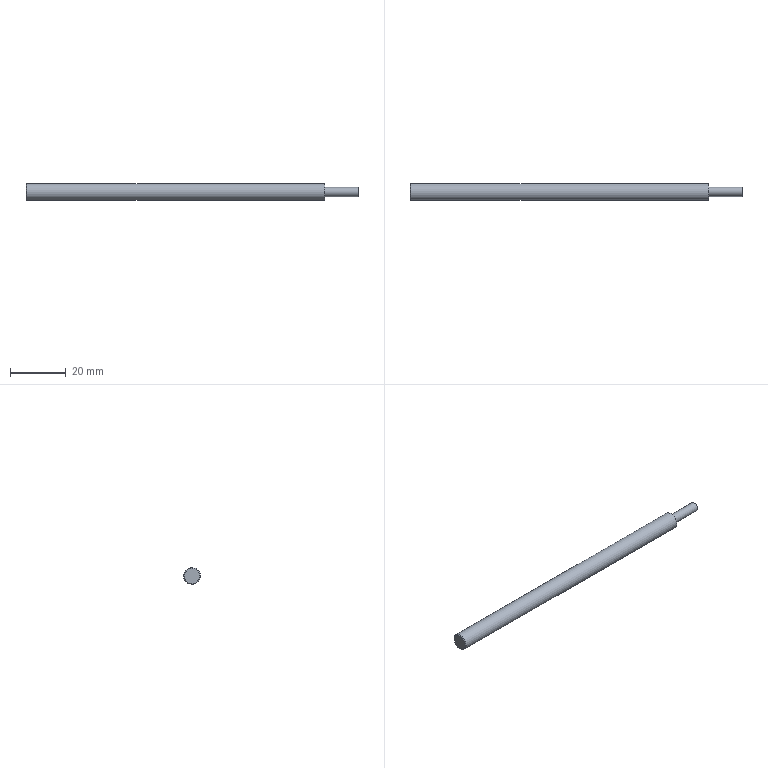Component | NX | PISTON_ROD | 1 solid | 6 faces | box 119 x 6 x 6 mm | volume 3127 mm3 | plane 3 | cylinder 2 | cone 1 | commonest cylinder face diameters 6 x1 3.3 x1
STEP:
#1=CARTESIAN_POINT('',(0.,0.,0.));
#2=DIRECTION('',(0.,0.,1.));
#3=DIRECTION('',(1.,0.,0.));
#4=AXIS2_PLACEMENT_3D('',#1,#2,#3);
#5=CARTESIAN_POINT('',(301.474,86.751,111.081));
#6=VERTEX_POINT('',#5);
#7=CARTESIAN_POINT('',(301.474,89.5,111.));
#8=DIRECTION('',(-1.,0.,0.));
#9=DIRECTION('',(0.,-0.9996,0.02941));
#10=AXIS2_PLACEMENT_3D('',#7,#8,#9);
#11=CIRCLE('',#10,2.75);
#12=CARTESIAN_POINT('',(301.474,89.5,111.));
#13=DIRECTION('',(-1.,0.,0.));
#14=DIRECTION('',(0.,-0.9996,0.02941));
#15=AXIS2_PLACEMENT_3D('',#12,#13,#14);
#16=PLANE('',#15);
#17=CARTESIAN_POINT('',(0.,0.));
#18=DIRECTION('',(1.,0.));
#19=AXIS2_PLACEMENT_2D('',#17,#18);
#20=CIRCLE('',#19,2.75);
#21=(GEOMETRIC_REPRESENTATION_CONTEXT(2)PARAMETRIC_REPRESENTATION_CONTEXT()REPRESENTATION_CONTEXT('',''));
#22=DEFINITIONAL_REPRESENTATION('',(#20),#21);
#23=PCURVE('',#16,#22);
#24=CARTESIAN_POINT('',(301.724,89.5,111.));
#25=DIRECTION('',(1.,0.,0.));
#26=DIRECTION('',(0.,0.9996,-0.02941));
#27=AXIS2_PLACEMENT_3D('',#24,#25,#26);
#28=CONICAL_SURFACE('',#27,3.,0.7854);
#29=CARTESIAN_POINT('',(9.425,-0.25));
#30=DIRECTION('',(-1.,0.));
#31=VECTOR('',#30,1.);
#32=LINE('',#29,#31);
#33=(GEOMETRIC_REPRESENTATION_CONTEXT(2)PARAMETRIC_REPRESENTATION_CONTEXT()REPRESENTATION_CONTEXT('',''));
#34=DEFINITIONAL_REPRESENTATION('',(#32),#33);
#35=PCURVE('',#28,#34);
#36=SURFACE_CURVE('',#11,(#23,#35),.PCURVE_S1.);
#37=EDGE_CURVE('',#6,#6,#36,.T.);
#38=ORIENTED_EDGE('',*,*,#37,.T.);
#39=EDGE_LOOP('',(#38));
#40=FACE_BOUND('',#39,.T.);
#41=ADVANCED_FACE('',(#40),#16,.T.);
#42=CARTESIAN_POINT('',(408.474,91.149,110.951));
#43=VERTEX_POINT('',#42);
#44=CARTESIAN_POINT('',(408.474,89.5,111.));
#45=DIRECTION('',(1.,0.,0.));
#46=DIRECTION('',(0.,0.9996,-0.02941));
#47=AXIS2_PLACEMENT_3D('',#44,#45,#46);
#48=CIRCLE('',#47,1.65);
#49=CARTESIAN_POINT('',(408.474,89.5,111.));
#50=DIRECTION('',(1.,0.,0.));
#51=DIRECTION('',(0.,0.9996,-0.02941));
#52=AXIS2_PLACEMENT_3D('',#49,#50,#51);
#53=PLANE('',#52);
#54=CARTESIAN_POINT('',(0.,0.));
#55=DIRECTION('',(1.,0.));
#56=AXIS2_PLACEMENT_2D('',#54,#55);
#57=CIRCLE('',#56,1.65);
#58=(GEOMETRIC_REPRESENTATION_CONTEXT(2)PARAMETRIC_REPRESENTATION_CONTEXT()REPRESENTATION_CONTEXT('',''));
#59=DEFINITIONAL_REPRESENTATION('',(#57),#58);
#60=PCURVE('',#53,#59);
#61=CARTESIAN_POINT('',(408.474,89.5,111.));
#62=DIRECTION('',(1.,0.,0.));
#63=DIRECTION('',(0.,0.9996,-0.02941));
#64=AXIS2_PLACEMENT_3D('',#61,#62,#63);
#65=CYLINDRICAL_SURFACE('',#64,1.65);
#66=CARTESIAN_POINT('',(0.,0.));
#67=DIRECTION('',(1.,0.));
#68=VECTOR('',#67,1.);
#69=LINE('',#66,#68);
#70=(GEOMETRIC_REPRESENTATION_CONTEXT(2)PARAMETRIC_REPRESENTATION_CONTEXT()REPRESENTATION_CONTEXT('',''));
#71=DEFINITIONAL_REPRESENTATION('',(#69),#70);
#72=PCURVE('',#65,#71);
#73=SURFACE_CURVE('',#48,(#60,#72),.PCURVE_S1.);
#74=EDGE_CURVE('',#43,#43,#73,.T.);
#75=ORIENTED_EDGE('',*,*,#74,.F.);
#76=EDGE_LOOP('',(#75));
#77=FACE_BOUND('',#76,.T.);
#78=CARTESIAN_POINT('',(408.474,86.501,111.088));
#79=VERTEX_POINT('',#78);
#80=CARTESIAN_POINT('',(408.474,89.5,111.));
#81=DIRECTION('',(-1.,0.,0.));
#82=DIRECTION('',(0.,-0.9996,0.02941));
#83=AXIS2_PLACEMENT_3D('',#80,#81,#82);
#84=CIRCLE('',#83,3.);
#85=CARTESIAN_POINT('',(-3.,-0.));
#86=CARTESIAN_POINT('',(-3.,5.196));
#87=CARTESIAN_POINT('',(1.5,2.598));
#88=CARTESIAN_POINT('',(6.,0.));
#89=CARTESIAN_POINT('',(1.5,-2.598));
#90=CARTESIAN_POINT('',(-3.,-5.196));
#91=CARTESIAN_POINT('',(-3.,-0.));
#92=(BOUNDED_CURVE()B_SPLINE_CURVE(2,(#85,#86,#87,#88,#89,#90,#91),.UNSPECIFIED.,.T.,.F.)B_SPLINE_CURVE_WITH_KNOTS((1,2,2,2,2,1),(-2.094,0.,2.094,4.189,6.283,8.378),.UNSPECIFIED.)CURVE()GEOMETRIC_REPRESENTATION_ITEM()RATIONAL_B_SPLINE_CURVE((1.,0.5,1.,0.5,1.,0.5,1.))REPRESENTATION_ITEM(''));
#93=(GEOMETRIC_REPRESENTATION_CONTEXT(2)PARAMETRIC_REPRESENTATION_CONTEXT()REPRESENTATION_CONTEXT('',''));
#94=DEFINITIONAL_REPRESENTATION('',(#92),#93);
#95=PCURVE('',#53,#94);
#96=CARTESIAN_POINT('',(408.474,89.5,111.));
#97=DIRECTION('',(-1.,0.,0.));
#98=DIRECTION('',(0.,-0.9996,0.02941));
#99=AXIS2_PLACEMENT_3D('',#96,#97,#98);
#100=CYLINDRICAL_SURFACE('',#99,3.);
#101=CARTESIAN_POINT('',(0.,0.));
#102=DIRECTION('',(1.,0.));
#103=VECTOR('',#102,1.);
#104=LINE('',#101,#103);
#105=(GEOMETRIC_REPRESENTATION_CONTEXT(2)PARAMETRIC_REPRESENTATION_CONTEXT()REPRESENTATION_CONTEXT('',''));
#106=DEFINITIONAL_REPRESENTATION('',(#104),#105);
#107=PCURVE('',#100,#106);
#108=SURFACE_CURVE('',#84,(#95,#107),.PCURVE_S1.);
#109=EDGE_CURVE('',#79,#79,#108,.T.);
#110=ORIENTED_EDGE('',*,*,#109,.F.);
#111=EDGE_LOOP('',(#110));
#112=FACE_BOUND('',#111,.T.);
#113=ADVANCED_FACE('',(#77,#112),#53,.T.);
#114=CARTESIAN_POINT('',(301.724,86.501,111.088));
#115=VERTEX_POINT('',#114);
#116=CARTESIAN_POINT('',(301.724,89.5,111.));
#117=DIRECTION('',(1.,0.,0.));
#118=DIRECTION('',(0.,-0.9996,0.02941));
#119=AXIS2_PLACEMENT_3D('',#116,#117,#118);
#120=CIRCLE('',#119,3.);
#121=CARTESIAN_POINT('',(6.283,106.75));
#122=DIRECTION('',(-1.,0.));
#123=VECTOR('',#122,1.);
#124=LINE('',#121,#123);
#125=(GEOMETRIC_REPRESENTATION_CONTEXT(2)PARAMETRIC_REPRESENTATION_CONTEXT()REPRESENTATION_CONTEXT('',''));
#126=DEFINITIONAL_REPRESENTATION('',(#124),#125);
#127=PCURVE('',#100,#126);
#128=CARTESIAN_POINT('',(3.142,0.));
#129=DIRECTION('',(1.,0.));
#130=VECTOR('',#129,1.);
#131=LINE('',#128,#130);
#132=(GEOMETRIC_REPRESENTATION_CONTEXT(2)PARAMETRIC_REPRESENTATION_CONTEXT()REPRESENTATION_CONTEXT('',''));
#133=DEFINITIONAL_REPRESENTATION('',(#131),#132);
#134=PCURVE('',#28,#133);
#135=SURFACE_CURVE('',#120,(#127,#134),.PCURVE_S1.);
#136=EDGE_CURVE('',#115,#115,#135,.T.);
#137=ORIENTED_EDGE('',*,*,#136,.T.);
#138=CARTESIAN_POINT('',(408.474,86.501,111.088));
#139=CARTESIAN_POINT('',(301.724,86.501,111.088));
#140=B_SPLINE_CURVE_WITH_KNOTS('',1,(#138,#139),.UNSPECIFIED.,.F.,.F.,(2,2),(0.,106.75),.PIECEWISE_BEZIER_KNOTS.);
#141=CARTESIAN_POINT('',(0.,0.));
#142=DIRECTION('',(0.,1.));
#143=VECTOR('',#142,1.);
#144=LINE('',#141,#143);
#145=(GEOMETRIC_REPRESENTATION_CONTEXT(2)PARAMETRIC_REPRESENTATION_CONTEXT()REPRESENTATION_CONTEXT('',''));
#146=DEFINITIONAL_REPRESENTATION('',(#144),#145);
#147=PCURVE('',#100,#146);
#148=CARTESIAN_POINT('',(6.283,0.));
#149=DIRECTION('',(0.,1.));
#150=VECTOR('',#149,1.);
#151=LINE('',#148,#150);
#152=(GEOMETRIC_REPRESENTATION_CONTEXT(2)PARAMETRIC_REPRESENTATION_CONTEXT()REPRESENTATION_CONTEXT('',''));
#153=DEFINITIONAL_REPRESENTATION('',(#151),#152);
#154=PCURVE('',#100,#153);
#155=SEAM_CURVE('',#140,(#147,#154),.PCURVE_S1.);
#156=EDGE_CURVE('',#79,#115,#155,.T.);
#157=ORIENTED_EDGE('',*,*,#156,.F.);
#158=ORIENTED_EDGE('',*,*,#109,.T.);
#159=ORIENTED_EDGE('',*,*,#156,.T.);
#160=EDGE_LOOP('',(#137,#157,#158,#159));
#161=FACE_BOUND('',#160,.T.);
#162=ADVANCED_FACE('',(#161),#100,.T.);
#163=CARTESIAN_POINT('',(420.474,91.149,110.951));
#164=VERTEX_POINT('',#163);
#165=CARTESIAN_POINT('',(420.474,89.5,111.));
#166=DIRECTION('',(1.,0.,0.));
#167=DIRECTION('',(0.,0.9996,-0.02941));
#168=AXIS2_PLACEMENT_3D('',#165,#166,#167);
#169=CIRCLE('',#168,1.65);
#170=CARTESIAN_POINT('',(420.474,89.5,111.));
#171=DIRECTION('',(1.,0.,0.));
#172=DIRECTION('',(0.,0.9996,-0.02941));
#173=AXIS2_PLACEMENT_3D('',#170,#171,#172);
#174=PLANE('',#173);
#175=CARTESIAN_POINT('',(0.,0.));
#176=DIRECTION('',(1.,0.));
#177=AXIS2_PLACEMENT_2D('',#175,#176);
#178=CIRCLE('',#177,1.65);
#179=(GEOMETRIC_REPRESENTATION_CONTEXT(2)PARAMETRIC_REPRESENTATION_CONTEXT()REPRESENTATION_CONTEXT('',''));
#180=DEFINITIONAL_REPRESENTATION('',(#178),#179);
#181=PCURVE('',#174,#180);
#182=CARTESIAN_POINT('',(0.,12.));
#183=DIRECTION('',(1.,0.));
#184=VECTOR('',#183,1.);
#185=LINE('',#182,#184);
#186=(GEOMETRIC_REPRESENTATION_CONTEXT(2)PARAMETRIC_REPRESENTATION_CONTEXT()REPRESENTATION_CONTEXT('',''));
#187=DEFINITIONAL_REPRESENTATION('',(#185),#186);
#188=PCURVE('',#65,#187);
#189=SURFACE_CURVE('',#169,(#181,#188),.PCURVE_S1.);
#190=EDGE_CURVE('',#164,#164,#189,.T.);
#191=ORIENTED_EDGE('',*,*,#190,.T.);
#192=EDGE_LOOP('',(#191));
#193=FACE_BOUND('',#192,.T.);
#194=ADVANCED_FACE('',(#193),#174,.T.);
#195=ORIENTED_EDGE('',*,*,#190,.F.);
#196=CARTESIAN_POINT('',(408.474,91.149,110.951));
#197=CARTESIAN_POINT('',(420.474,91.149,110.951));
#198=B_SPLINE_CURVE_WITH_KNOTS('',1,(#196,#197),.UNSPECIFIED.,.F.,.F.,(2,2),(0.,12.),.PIECEWISE_BEZIER_KNOTS.);
#199=CARTESIAN_POINT('',(0.,0.));
#200=DIRECTION('',(0.,1.));
#201=VECTOR('',#200,1.);
#202=LINE('',#199,#201);
#203=(GEOMETRIC_REPRESENTATION_CONTEXT(2)PARAMETRIC_REPRESENTATION_CONTEXT()REPRESENTATION_CONTEXT('',''));
#204=DEFINITIONAL_REPRESENTATION('',(#202),#203);
#205=PCURVE('',#65,#204);
#206=CARTESIAN_POINT('',(6.283,0.));
#207=DIRECTION('',(0.,1.));
#208=VECTOR('',#207,1.);
#209=LINE('',#206,#208);
#210=(GEOMETRIC_REPRESENTATION_CONTEXT(2)PARAMETRIC_REPRESENTATION_CONTEXT()REPRESENTATION_CONTEXT('',''));
#211=DEFINITIONAL_REPRESENTATION('',(#209),#210);
#212=PCURVE('',#65,#211);
#213=SEAM_CURVE('',#198,(#205,#212),.PCURVE_S1.);
#214=EDGE_CURVE('',#43,#164,#213,.T.);
#215=ORIENTED_EDGE('',*,*,#214,.F.);
#216=ORIENTED_EDGE('',*,*,#74,.T.);
#217=ORIENTED_EDGE('',*,*,#214,.T.);
#218=EDGE_LOOP('',(#195,#215,#216,#217));
#219=FACE_BOUND('',#218,.T.);
#220=ADVANCED_FACE('',(#219),#65,.T.);
#221=ORIENTED_EDGE('',*,*,#37,.F.);
#222=CARTESIAN_POINT('',(301.474,86.751,111.081));
#223=CARTESIAN_POINT('',(301.724,86.501,111.088));
#224=B_SPLINE_CURVE_WITH_KNOTS('',1,(#222,#223),.UNSPECIFIED.,.F.,.F.,(2,2),(-0.3536,0.),.PIECEWISE_BEZIER_KNOTS.);
#225=CARTESIAN_POINT('',(9.425,0.));
#226=DIRECTION('',(0.,1.));
#227=VECTOR('',#226,1.);
#228=LINE('',#225,#227);
#229=(GEOMETRIC_REPRESENTATION_CONTEXT(2)PARAMETRIC_REPRESENTATION_CONTEXT()REPRESENTATION_CONTEXT('',''));
#230=DEFINITIONAL_REPRESENTATION('',(#228),#229);
#231=PCURVE('',#28,#230);
#232=CARTESIAN_POINT('',(3.142,0.));
#233=DIRECTION('',(0.,1.));
#234=VECTOR('',#233,1.);
#235=LINE('',#232,#234);
#236=(GEOMETRIC_REPRESENTATION_CONTEXT(2)PARAMETRIC_REPRESENTATION_CONTEXT()REPRESENTATION_CONTEXT('',''));
#237=DEFINITIONAL_REPRESENTATION('',(#235),#236);
#238=PCURVE('',#28,#237);
#239=SEAM_CURVE('',#224,(#231,#238),.PCURVE_S1.);
#240=EDGE_CURVE('',#6,#115,#239,.T.);
#241=ORIENTED_EDGE('',*,*,#240,.T.);
#242=ORIENTED_EDGE('',*,*,#136,.F.);
#243=ORIENTED_EDGE('',*,*,#240,.F.);
#244=EDGE_LOOP('',(#221,#241,#242,#243));
#245=FACE_BOUND('',#244,.T.);
#246=ADVANCED_FACE('',(#245),#28,.T.);
#247=CLOSED_SHELL('',(#41,#113,#162,#194,#220,#246));
#248=MANIFOLD_SOLID_BREP('',#247);
#249=(LENGTH_UNIT()NAMED_UNIT(*)SI_UNIT(.MILLI.,.METRE.));
#250=UNCERTAINTY_MEASURE_WITH_UNIT(LENGTH_MEASURE(0.00001),#249,'','');
#251=(NAMED_UNIT(*)PLANE_ANGLE_UNIT()SI_UNIT($,.RADIAN.));
#252=(NAMED_UNIT(*)SI_UNIT($,.STERADIAN.)SOLID_ANGLE_UNIT());
#253=(GEOMETRIC_REPRESENTATION_CONTEXT(3)GLOBAL_UNCERTAINTY_ASSIGNED_CONTEXT((#250))GLOBAL_UNIT_ASSIGNED_CONTEXT((#249,#251,#252))REPRESENTATION_CONTEXT('',''));
#254=ADVANCED_BREP_SHAPE_REPRESENTATION('',(#4,#248),#253);